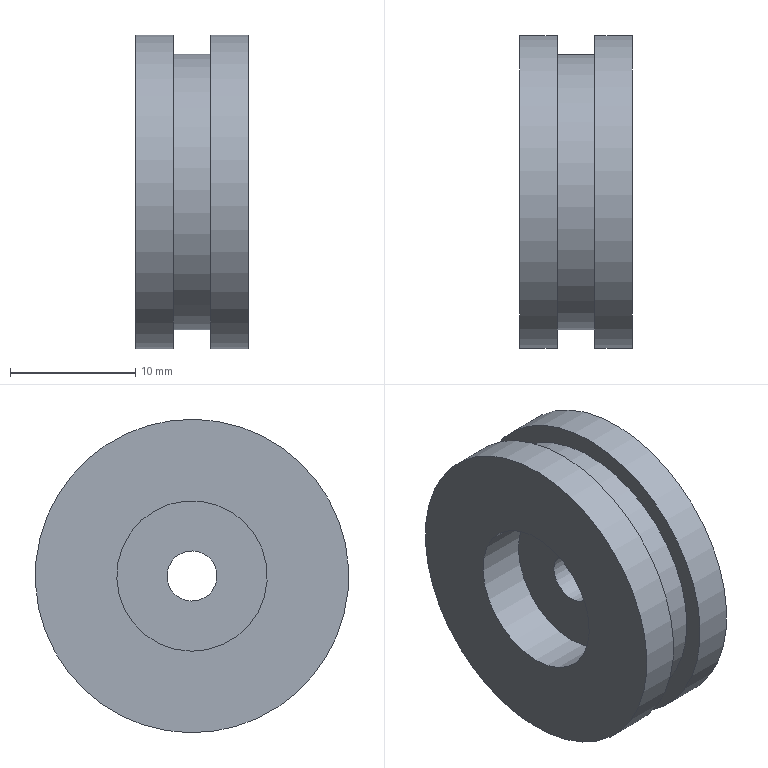Component | NX | PISTON | 1 solid | 12 faces | volume 3556 mm3 | cylinder 6 | plane 6 | commonest cylinder face diameters 25 x2 4 x1 22 x1 5 x1 12 x1